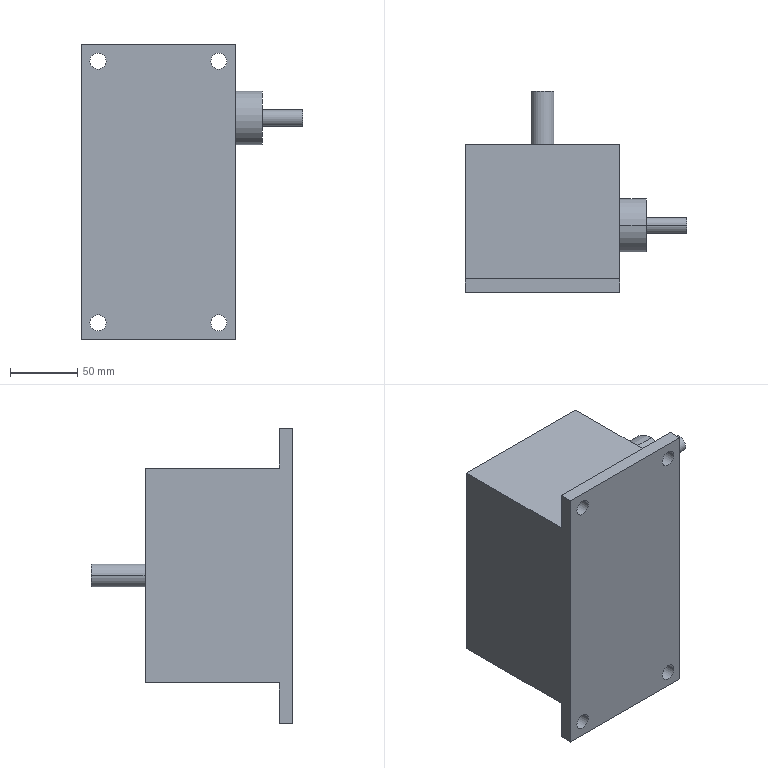Component | SolidWorks | Motor2-1 | 1 solid | 27 faces | box 165 x 150 x 220 mm | volume 2126081 mm3 | cylinder 14 | plane 13 | commonest cylinder face diameters 12 x10 40 x2 17 x2
build123d program:
from build123d import *

# Parameters (mm, degrees)
SKETCH1_W      = 220
SKETCH1_H      = 115
SKETCH1_R      = 6
EXTRUDE1_DEPTH = 10
SKETCH2_W      = 160
SKETCH2_H      = 115
EXTRUDE2_DEPTH = 100
SKETCH4_R      = 8.5
EXTRUDE3_DEPTH = 40
SKETCH5_R      = 20
EXTRUDE4_DEPTH = 20
SKETCH6_R      = 6
EXTRUDE5_DEPTH = 30


with BuildPart() as part:
    # Sketch1 → Extrude1 (new body)
    with BuildSketch(Plane(origin=(0, 0, 0), x_dir=(1, 0, 0), z_dir=(0, 1, 0))):
        with Locations((71.152, -39.253)):
            Rectangle(SKETCH1_W, SKETCH1_H)
        with Locations(Location((-26.348, 5.747, 0), (0, 0, 270))):
            Circle(SKETCH1_R, mode=Mode.SUBTRACT)
        with Locations(Location((168.652, 5.747, 0), (0, 0, 270))):
            Circle(SKETCH1_R, mode=Mode.SUBTRACT)
        with Locations(Location((-26.348, -84.253, 0), (0, 0, 270))):
            Circle(SKETCH1_R, mode=Mode.SUBTRACT)
        with Locations(Location((168.652, -84.253, 0), (0, 0, 270))):
            Circle(SKETCH1_R, mode=Mode.SUBTRACT)
    extrude(amount=EXTRUDE1_DEPTH)

    # Sketch2 → Extrude2 (add)
    with BuildSketch(Plane(origin=(0, 10, 0), x_dir=(1, 0, 0), z_dir=(0, 1, 0))):
        with Locations((70.757, -39.253)):
            Rectangle(SKETCH2_W, SKETCH2_H)
    extrude(amount=EXTRUDE2_DEPTH)

    # Sketch4 → Extrude3 (add)
    with BuildSketch(Plane(origin=(0, 110, 0), x_dir=(-1, 0, 0), z_dir=(0, 1, 0))):
        with Locations(Location((-70.757, 39.253, 0), (0, 0, 90))):
            Circle(SKETCH4_R)
    extrude(amount=EXTRUDE3_DEPTH)

    # Sketch5 → Extrude4 (add)
    with BuildSketch(Plane.XY.offset(96.753)):
        with Locations(Location((16.02, 50, 0), (0, 0, 180))):
            Circle(SKETCH5_R)
    extrude(amount=EXTRUDE4_DEPTH)

    # Sketch6 → Extrude5 (add)
    with BuildSketch(Plane.XY.offset(116.753)):
        with Locations((16.02, 50)):
            Circle(SKETCH6_R)
    extrude(amount=EXTRUDE5_DEPTH)


solid = part.part

# Placed as in the assembly
solid = solid.moved(Location((-204.037, 125.983, 74.757), (0, 90, 0)))
STEP:
#1=COLOUR_RGB('',0.7922,0.8196,0.9333);
#2=FILL_AREA_STYLE_COLOUR('',#1);
#3=FILL_AREA_STYLE('',(#2));
#4=SURFACE_STYLE_FILL_AREA(#3);
#5=SURFACE_SIDE_STYLE('',(#4));
#6=SURFACE_STYLE_USAGE(.BOTH.,#5);
#7=PRESENTATION_STYLE_ASSIGNMENT((#6));
#8=CARTESIAN_POINT('',(-2.255,6.928,2.076));
#9=VERTEX_POINT('',#8);
#10=CARTESIAN_POINT('',(-2.255,6.928,2.549));
#11=VERTEX_POINT('',#10);
#12=CARTESIAN_POINT('',(-2.255,6.928,2.312));
#13=DIRECTION('',(1.,0.,0.));
#14=DIRECTION('',(0.,0.,-1.));
#15=AXIS2_PLACEMENT_3D('',#12,#13,#14);
#16=CIRCLE('',#15,0.2362);
#17=EDGE_CURVE('',#9,#11,#16,.T.);
#18=ORIENTED_EDGE('',*,*,#17,.F.);
#19=CARTESIAN_POINT('',(-3.436,6.928,2.076));
#20=VERTEX_POINT('',#19);
#21=CARTESIAN_POINT('',(-2.255,6.928,2.076));
#22=DIRECTION('',(-1.,-0.,-0.));
#23=VECTOR('',#22,39.37);
#24=LINE('',#21,#23);
#25=EDGE_CURVE('',#9,#20,#24,.T.);
#26=ORIENTED_EDGE('',*,*,#25,.T.);
#27=CARTESIAN_POINT('',(-3.436,6.928,2.549));
#28=VERTEX_POINT('',#27);
#29=CARTESIAN_POINT('',(-3.436,6.928,2.312));
#30=DIRECTION('',(1.,0.,0.));
#31=DIRECTION('',(0.,0.,-1.));
#32=AXIS2_PLACEMENT_3D('',#29,#30,#31);
#33=CIRCLE('',#32,0.2362);
#34=EDGE_CURVE('',#20,#28,#33,.T.);
#35=ORIENTED_EDGE('',*,*,#34,.T.);
#36=CARTESIAN_POINT('',(-2.255,6.928,2.549));
#37=DIRECTION('',(-1.,-0.,-0.));
#38=VECTOR('',#37,39.37);
#39=LINE('',#36,#38);
#40=EDGE_CURVE('',#11,#28,#39,.T.);
#41=ORIENTED_EDGE('',*,*,#40,.F.);
#42=EDGE_LOOP('',(#18,#26,#35,#41));
#43=FACE_OUTER_BOUND('',#42,.T.);
#44=CARTESIAN_POINT('',(-2.255,6.928,2.312));
#45=DIRECTION('',(-1.,-0.,-0.));
#46=DIRECTION('',(0.,0.,1.));
#47=AXIS2_PLACEMENT_3D('',#44,#45,#46);
#48=CYLINDRICAL_SURFACE('',#47,0.2362);
#49=ADVANCED_FACE('',(#43),#48,.T.);
#50=CARTESIAN_POINT('',(-3.436,6.928,1.525));
#51=VERTEX_POINT('',#50);
#52=CARTESIAN_POINT('',(-3.436,6.928,3.1));
#53=VERTEX_POINT('',#52);
#54=CARTESIAN_POINT('',(-3.436,6.928,2.312));
#55=DIRECTION('',(1.,0.,0.));
#56=DIRECTION('',(0.,0.,-1.));
#57=AXIS2_PLACEMENT_3D('',#54,#55,#56);
#58=CIRCLE('',#57,0.7874);
#59=EDGE_CURVE('',#51,#53,#58,.T.);
#60=ORIENTED_EDGE('',*,*,#59,.F.);
#61=CARTESIAN_POINT('',(-4.224,6.928,1.525));
#62=VERTEX_POINT('',#61);
#63=CARTESIAN_POINT('',(-3.436,6.928,1.525));
#64=DIRECTION('',(-1.,-0.,-0.));
#65=VECTOR('',#64,39.37);
#66=LINE('',#63,#65);
#67=EDGE_CURVE('',#51,#62,#66,.T.);
#68=ORIENTED_EDGE('',*,*,#67,.T.);
#69=CARTESIAN_POINT('',(-4.224,6.928,3.1));
#70=VERTEX_POINT('',#69);
#71=CARTESIAN_POINT('',(-4.224,6.928,2.312));
#72=DIRECTION('',(1.,0.,0.));
#73=DIRECTION('',(0.,0.,1.));
#74=AXIS2_PLACEMENT_3D('',#71,#72,#73);
#75=CIRCLE('',#74,0.7874);
#76=EDGE_CURVE('',#62,#70,#75,.T.);
#77=ORIENTED_EDGE('',*,*,#76,.T.);
#78=CARTESIAN_POINT('',(-3.436,6.928,3.1));
#79=DIRECTION('',(-1.,-0.,-0.));
#80=VECTOR('',#79,39.37);
#81=LINE('',#78,#80);
#82=EDGE_CURVE('',#53,#70,#81,.T.);
#83=ORIENTED_EDGE('',*,*,#82,.F.);
#84=EDGE_LOOP('',(#60,#68,#77,#83));
#85=FACE_OUTER_BOUND('',#84,.T.);
#86=CARTESIAN_POINT('',(-3.436,6.928,2.312));
#87=DIRECTION('',(-1.,-0.,-0.));
#88=DIRECTION('',(0.,0.,1.));
#89=AXIS2_PLACEMENT_3D('',#86,#87,#88);
#90=CYLINDRICAL_SURFACE('',#89,0.7874);
#91=ADVANCED_FACE('',(#85),#90,.T.);
#92=CARTESIAN_POINT('',(-6.153,10.865,0.1575));
#93=VERTEX_POINT('',#92);
#94=CARTESIAN_POINT('',(-6.822,10.865,0.1575));
#95=VERTEX_POINT('',#94);
#96=CARTESIAN_POINT('',(-6.488,10.865,0.1575));
#97=DIRECTION('',(-0.,1.,-0.));
#98=DIRECTION('',(1.,0.,0.));
#99=AXIS2_PLACEMENT_3D('',#96,#97,#98);
#100=CIRCLE('',#99,0.3346);
#101=EDGE_CURVE('',#93,#95,#100,.T.);
#102=ORIENTED_EDGE('',*,*,#101,.F.);
#103=CARTESIAN_POINT('',(-6.153,9.291,0.1575));
#104=VERTEX_POINT('',#103);
#105=CARTESIAN_POINT('',(-6.153,10.865,0.1575));
#106=DIRECTION('',(0.,-1.,0.));
#107=VECTOR('',#106,39.37);
#108=LINE('',#105,#107);
#109=EDGE_CURVE('',#93,#104,#108,.T.);
#110=ORIENTED_EDGE('',*,*,#109,.T.);
#111=CARTESIAN_POINT('',(-6.822,9.291,0.1575));
#112=VERTEX_POINT('',#111);
#113=CARTESIAN_POINT('',(-6.488,9.291,0.1575));
#114=DIRECTION('',(-0.,1.,-0.));
#115=DIRECTION('',(1.,0.,0.));
#116=AXIS2_PLACEMENT_3D('',#113,#114,#115);
#117=CIRCLE('',#116,0.3346);
#118=EDGE_CURVE('',#104,#112,#117,.T.);
#119=ORIENTED_EDGE('',*,*,#118,.T.);
#120=CARTESIAN_POINT('',(-6.822,10.865,0.1575));
#121=DIRECTION('',(0.,-1.,0.));
#122=VECTOR('',#121,39.37);
#123=LINE('',#120,#122);
#124=EDGE_CURVE('',#95,#112,#123,.T.);
#125=ORIENTED_EDGE('',*,*,#124,.F.);
#126=EDGE_LOOP('',(#102,#110,#119,#125));
#127=FACE_OUTER_BOUND('',#126,.T.);
#128=CARTESIAN_POINT('',(-6.488,10.865,0.1575));
#129=DIRECTION('',(0.,-1.,0.));
#130=DIRECTION('',(-1.,0.,-0.));
#131=AXIS2_PLACEMENT_3D('',#128,#129,#130);
#132=CYLINDRICAL_SURFACE('',#131,0.3346);
#133=ADVANCED_FACE('',(#127),#132,.T.);
#134=CARTESIAN_POINT('',(-4.952,5.354,-3.697));
#135=VERTEX_POINT('',#134);
#136=CARTESIAN_POINT('',(-4.48,5.354,-3.697));
#137=VERTEX_POINT('',#136);
#138=CARTESIAN_POINT('',(-4.716,5.354,-3.697));
#139=DIRECTION('',(-0.,1.,-0.));
#140=DIRECTION('',(1.,0.,0.));
#141=AXIS2_PLACEMENT_3D('',#138,#139,#140);
#142=CIRCLE('',#141,0.2362);
#143=EDGE_CURVE('',#135,#137,#142,.T.);
#144=ORIENTED_EDGE('',*,*,#143,.T.);
#145=CARTESIAN_POINT('',(-4.48,4.96,-3.697));
#146=VERTEX_POINT('',#145);
#147=CARTESIAN_POINT('',(-4.48,5.354,-3.697));
#148=DIRECTION('',(0.,-1.,0.));
#149=VECTOR('',#148,39.37);
#150=LINE('',#147,#149);
#151=EDGE_CURVE('',#137,#146,#150,.T.);
#152=ORIENTED_EDGE('',*,*,#151,.T.);
#153=CARTESIAN_POINT('',(-4.952,4.96,-3.697));
#154=VERTEX_POINT('',#153);
#155=CARTESIAN_POINT('',(-4.716,4.96,-3.697));
#156=DIRECTION('',(-0.,1.,-0.));
#157=DIRECTION('',(1.,0.,0.));
#158=AXIS2_PLACEMENT_3D('',#155,#156,#157);
#159=CIRCLE('',#158,0.2362);
#160=EDGE_CURVE('',#154,#146,#159,.T.);
#161=ORIENTED_EDGE('',*,*,#160,.F.);
#162=CARTESIAN_POINT('',(-4.952,5.354,-3.697));
#163=DIRECTION('',(0.,-1.,0.));
#164=VECTOR('',#163,39.37);
#165=LINE('',#162,#164);
#166=EDGE_CURVE('',#135,#154,#165,.T.);
#167=ORIENTED_EDGE('',*,*,#166,.F.);
#168=EDGE_LOOP('',(#144,#152,#161,#167));
#169=FACE_OUTER_BOUND('',#168,.T.);
#170=CARTESIAN_POINT('',(-4.716,5.354,-3.697));
#171=DIRECTION('',(0.,-1.,0.));
#172=DIRECTION('',(-1.,0.,0.));
#173=AXIS2_PLACEMENT_3D('',#170,#171,#172);
#174=CYLINDRICAL_SURFACE('',#173,0.2362);
#175=ADVANCED_FACE('',(#169),#174,.F.);
#176=CARTESIAN_POINT('',(-4.952,5.354,3.98));
#177=VERTEX_POINT('',#176);
#178=CARTESIAN_POINT('',(-4.48,5.354,3.98));
#179=VERTEX_POINT('',#178);
#180=CARTESIAN_POINT('',(-4.716,5.354,3.98));
#181=DIRECTION('',(-0.,1.,-0.));
#182=DIRECTION('',(1.,0.,0.));
#183=AXIS2_PLACEMENT_3D('',#180,#181,#182);
#184=CIRCLE('',#183,0.2362);
#185=EDGE_CURVE('',#177,#179,#184,.T.);
#186=ORIENTED_EDGE('',*,*,#185,.T.);
#187=CARTESIAN_POINT('',(-4.48,4.96,3.98));
#188=VERTEX_POINT('',#187);
#189=CARTESIAN_POINT('',(-4.48,5.354,3.98));
#190=DIRECTION('',(0.,-1.,0.));
#191=VECTOR('',#190,39.37);
#192=LINE('',#189,#191);
#193=EDGE_CURVE('',#179,#188,#192,.T.);
#194=ORIENTED_EDGE('',*,*,#193,.T.);
#195=CARTESIAN_POINT('',(-4.952,4.96,3.98));
#196=VERTEX_POINT('',#195);
#197=CARTESIAN_POINT('',(-4.716,4.96,3.98));
#198=DIRECTION('',(-0.,1.,-0.));
#199=DIRECTION('',(1.,0.,0.));
#200=AXIS2_PLACEMENT_3D('',#197,#198,#199);
#201=CIRCLE('',#200,0.2362);
#202=EDGE_CURVE('',#196,#188,#201,.T.);
#203=ORIENTED_EDGE('',*,*,#202,.F.);
#204=CARTESIAN_POINT('',(-4.952,5.354,3.98));
#205=DIRECTION('',(0.,-1.,0.));
#206=VECTOR('',#205,39.37);
#207=LINE('',#204,#206);
#208=EDGE_CURVE('',#177,#196,#207,.T.);
#209=ORIENTED_EDGE('',*,*,#208,.F.);
#210=EDGE_LOOP('',(#186,#194,#203,#209));
#211=FACE_OUTER_BOUND('',#210,.T.);
#212=CARTESIAN_POINT('',(-4.716,5.354,3.98));
#213=DIRECTION('',(0.,-1.,0.));
#214=DIRECTION('',(-1.,0.,0.));
#215=AXIS2_PLACEMENT_3D('',#212,#213,#214);
#216=CYLINDRICAL_SURFACE('',#215,0.2362);
#217=ADVANCED_FACE('',(#211),#216,.F.);
#218=CARTESIAN_POINT('',(-8.495,5.354,-3.697));
#219=VERTEX_POINT('',#218);
#220=CARTESIAN_POINT('',(-8.023,5.354,-3.697));
#221=VERTEX_POINT('',#220);
#222=CARTESIAN_POINT('',(-8.259,5.354,-3.697));
#223=DIRECTION('',(-0.,1.,-0.));
#224=DIRECTION('',(1.,0.,0.));
#225=AXIS2_PLACEMENT_3D('',#222,#223,#224);
#226=CIRCLE('',#225,0.2362);
#227=EDGE_CURVE('',#219,#221,#226,.T.);
#228=ORIENTED_EDGE('',*,*,#227,.T.);
#229=CARTESIAN_POINT('',(-8.023,4.96,-3.697));
#230=VERTEX_POINT('',#229);
#231=CARTESIAN_POINT('',(-8.023,5.354,-3.697));
#232=DIRECTION('',(0.,-1.,0.));
#233=VECTOR('',#232,39.37);
#234=LINE('',#231,#233);
#235=EDGE_CURVE('',#221,#230,#234,.T.);
#236=ORIENTED_EDGE('',*,*,#235,.T.);
#237=CARTESIAN_POINT('',(-8.495,4.96,-3.697));
#238=VERTEX_POINT('',#237);
#239=CARTESIAN_POINT('',(-8.259,4.96,-3.697));
#240=DIRECTION('',(-0.,1.,-0.));
#241=DIRECTION('',(1.,0.,0.));
#242=AXIS2_PLACEMENT_3D('',#239,#240,#241);
#243=CIRCLE('',#242,0.2362);
#244=EDGE_CURVE('',#238,#230,#243,.T.);
#245=ORIENTED_EDGE('',*,*,#244,.F.);
#246=CARTESIAN_POINT('',(-8.495,5.354,-3.697));
#247=DIRECTION('',(0.,-1.,0.));
#248=VECTOR('',#247,39.37);
#249=LINE('',#246,#248);
#250=EDGE_CURVE('',#219,#238,#249,.T.);
#251=ORIENTED_EDGE('',*,*,#250,.F.);
#252=EDGE_LOOP('',(#228,#236,#245,#251));
#253=FACE_OUTER_BOUND('',#252,.T.);
#254=CARTESIAN_POINT('',(-8.259,5.354,-3.697));
#255=DIRECTION('',(0.,-1.,0.));
#256=DIRECTION('',(-1.,0.,0.));
#257=AXIS2_PLACEMENT_3D('',#254,#255,#256);
#258=CYLINDRICAL_SURFACE('',#257,0.2362);
#259=ADVANCED_FACE('',(#253),#258,.F.);
#260=CARTESIAN_POINT('',(-8.495,5.354,3.98));
#261=VERTEX_POINT('',#260);
#262=CARTESIAN_POINT('',(-8.023,5.354,3.98));
#263=VERTEX_POINT('',#262);
#264=CARTESIAN_POINT('',(-8.259,5.354,3.98));
#265=DIRECTION('',(-0.,1.,-0.));
#266=DIRECTION('',(1.,0.,0.));
#267=AXIS2_PLACEMENT_3D('',#264,#265,#266);
#268=CIRCLE('',#267,0.2362);
#269=EDGE_CURVE('',#261,#263,#268,.T.);
#270=ORIENTED_EDGE('',*,*,#269,.T.);
#271=CARTESIAN_POINT('',(-8.023,4.96,3.98));
#272=VERTEX_POINT('',#271);
#273=CARTESIAN_POINT('',(-8.023,5.354,3.98));
#274=DIRECTION('',(0.,-1.,0.));
#275=VECTOR('',#274,39.37);
#276=LINE('',#273,#275);
#277=EDGE_CURVE('',#263,#272,#276,.T.);
#278=ORIENTED_EDGE('',*,*,#277,.T.);
#279=CARTESIAN_POINT('',(-8.495,4.96,3.98));
#280=VERTEX_POINT('',#279);
#281=CARTESIAN_POINT('',(-8.259,4.96,3.98));
#282=DIRECTION('',(-0.,1.,-0.));
#283=DIRECTION('',(1.,0.,0.));
#284=AXIS2_PLACEMENT_3D('',#281,#282,#283);
#285=CIRCLE('',#284,0.2362);
#286=EDGE_CURVE('',#280,#272,#285,.T.);
#287=ORIENTED_EDGE('',*,*,#286,.F.);
#288=CARTESIAN_POINT('',(-8.495,5.354,3.98));
#289=DIRECTION('',(0.,-1.,0.));
#290=VECTOR('',#289,39.37);
#291=LINE('',#288,#290);
#292=EDGE_CURVE('',#261,#280,#291,.T.);
#293=ORIENTED_EDGE('',*,*,#292,.F.);
#294=EDGE_LOOP('',(#270,#278,#287,#293));
#295=FACE_OUTER_BOUND('',#294,.T.);
#296=CARTESIAN_POINT('',(-8.259,5.354,3.98));
#297=DIRECTION('',(0.,-1.,0.));
#298=DIRECTION('',(-1.,0.,0.));
#299=AXIS2_PLACEMENT_3D('',#296,#297,#298);
#300=CYLINDRICAL_SURFACE('',#299,0.2362);
#301=ADVANCED_FACE('',(#295),#300,.F.);
#302=CARTESIAN_POINT('',(-3.436,6.928,2.312));
#303=DIRECTION('',(1.,0.,0.));
#304=DIRECTION('',(0.,0.,-1.));
#305=AXIS2_PLACEMENT_3D('',#302,#303,#304);
#306=CIRCLE('',#305,0.7874);
#307=EDGE_CURVE('',#53,#51,#306,.T.);
#308=ORIENTED_EDGE('',*,*,#307,.T.);
#309=ORIENTED_EDGE('',*,*,#59,.T.);
#310=EDGE_LOOP('',(#308,#309));
#311=FACE_OUTER_BOUND('',#310,.T.);
#312=CARTESIAN_POINT('',(-3.436,6.928,2.312));
#313=DIRECTION('',(1.,0.,0.));
#314=DIRECTION('',(0.,0.,-1.));
#315=AXIS2_PLACEMENT_3D('',#312,#313,#314);
#316=CIRCLE('',#315,0.2362);
#317=EDGE_CURVE('',#28,#20,#316,.T.);
#318=ORIENTED_EDGE('',*,*,#317,.F.);
#319=ORIENTED_EDGE('',*,*,#34,.F.);
#320=EDGE_LOOP('',(#318,#319));
#321=FACE_BOUND('',#320,.T.);
#322=CARTESIAN_POINT('',(-3.436,6.928,2.312));
#323=DIRECTION('',(1.,0.,0.));
#324=DIRECTION('',(0.,-0.,-1.));
#325=AXIS2_PLACEMENT_3D('',#322,#323,#324);
#326=PLANE('',#325);
#327=ADVANCED_FACE('',(#311,#321),#326,.T.);
#328=CARTESIAN_POINT('',(-4.224,4.96,4.473));
#329=VERTEX_POINT('',#328);
#330=CARTESIAN_POINT('',(-4.224,4.96,-4.189));
#331=VERTEX_POINT('',#330);
#332=CARTESIAN_POINT('',(-4.224,4.96,4.473));
#333=DIRECTION('',(0.,-0.,-1.));
#334=VECTOR('',#333,39.37);
#335=LINE('',#332,#334);
#336=EDGE_CURVE('',#329,#331,#335,.T.);
#337=ORIENTED_EDGE('',*,*,#336,.T.);
#338=CARTESIAN_POINT('',(-4.224,5.354,-4.189));
#339=VERTEX_POINT('',#338);
#340=CARTESIAN_POINT('',(-4.224,5.354,-4.189));
#341=DIRECTION('',(0.,-1.,0.));
#342=VECTOR('',#341,39.37);
#343=LINE('',#340,#342);
#344=EDGE_CURVE('',#339,#331,#343,.T.);
#345=ORIENTED_EDGE('',*,*,#344,.F.);
#346=CARTESIAN_POINT('',(-4.224,5.354,-2.992));
#347=VERTEX_POINT('',#346);
#348=CARTESIAN_POINT('',(-4.224,5.354,4.473));
#349=DIRECTION('',(0.,-0.,-1.));
#350=VECTOR('',#349,39.37);
#351=LINE('',#348,#350);
#352=EDGE_CURVE('',#347,#339,#351,.T.);
#353=ORIENTED_EDGE('',*,*,#352,.F.);
#354=CARTESIAN_POINT('',(-4.224,9.291,-2.992));
#355=VERTEX_POINT('',#354);
#356=CARTESIAN_POINT('',(-4.224,9.291,-2.992));
#357=DIRECTION('',(0.,-1.,0.));
#358=VECTOR('',#357,39.37);
#359=LINE('',#356,#358);
#360=EDGE_CURVE('',#355,#347,#359,.T.);
#361=ORIENTED_EDGE('',*,*,#360,.F.);
#362=CARTESIAN_POINT('',(-4.224,9.291,3.307));
#363=VERTEX_POINT('',#362);
#364=CARTESIAN_POINT('',(-4.224,9.291,3.307));
#365=DIRECTION('',(0.,-0.,-1.));
#366=VECTOR('',#365,39.37);
#367=LINE('',#364,#366);
#368=EDGE_CURVE('',#363,#355,#367,.T.);
#369=ORIENTED_EDGE('',*,*,#368,.F.);
#370=CARTESIAN_POINT('',(-4.224,5.354,3.307));
#371=VERTEX_POINT('',#370);
#372=CARTESIAN_POINT('',(-4.224,9.291,3.307));
#373=DIRECTION('',(0.,-1.,0.));
#374=VECTOR('',#373,39.37);
#375=LINE('',#372,#374);
#376=EDGE_CURVE('',#363,#371,#375,.T.);
#377=ORIENTED_EDGE('',*,*,#376,.T.);
#378=CARTESIAN_POINT('',(-4.224,5.354,4.473));
#379=VERTEX_POINT('',#378);
#380=CARTESIAN_POINT('',(-4.224,5.354,4.473));
#381=DIRECTION('',(0.,-0.,-1.));
#382=VECTOR('',#381,39.37);
#383=LINE('',#380,#382);
#384=EDGE_CURVE('',#379,#371,#383,.T.);
#385=ORIENTED_EDGE('',*,*,#384,.F.);
#386=CARTESIAN_POINT('',(-4.224,5.354,4.473));
#387=DIRECTION('',(0.,-1.,0.));
#388=VECTOR('',#387,39.37);
#389=LINE('',#386,#388);
#390=EDGE_CURVE('',#379,#329,#389,.T.);
#391=ORIENTED_EDGE('',*,*,#390,.T.);
#392=EDGE_LOOP('',(#337,#345,#353,#361,#369,#377,#385,#391));
#393=FACE_OUTER_BOUND('',#392,.T.);
#394=CARTESIAN_POINT('',(-4.224,6.928,2.312));
#395=DIRECTION('',(1.,0.,0.));
#396=DIRECTION('',(0.,0.,1.));
#397=AXIS2_PLACEMENT_3D('',#394,#395,#396);
#398=CIRCLE('',#397,0.7874);
#399=EDGE_CURVE('',#70,#62,#398,.T.);
#400=ORIENTED_EDGE('',*,*,#399,.F.);
#401=ORIENTED_EDGE('',*,*,#76,.F.);
#402=EDGE_LOOP('',(#400,#401));
#403=FACE_BOUND('',#402,.T.);
#404=CARTESIAN_POINT('',(-4.224,5.354,4.473));
#405=DIRECTION('',(-1.,-0.,-0.));
#406=DIRECTION('',(-0.,0.,1.));
#407=AXIS2_PLACEMENT_3D('',#404,#405,#406);
#408=PLANE('',#407);
#409=ADVANCED_FACE('',(#393,#403),#408,.F.);
#410=CARTESIAN_POINT('',(-8.751,9.291,3.307));
#411=VERTEX_POINT('',#410);
#412=CARTESIAN_POINT('',(-8.751,9.291,3.307));
#413=DIRECTION('',(1.,0.,0.));
#414=VECTOR('',#413,39.37);
#415=LINE('',#412,#414);
#416=EDGE_CURVE('',#411,#363,#415,.T.);
#417=ORIENTED_EDGE('',*,*,#416,.T.);
#418=ORIENTED_EDGE('',*,*,#368,.T.);
#419=CARTESIAN_POINT('',(-8.751,9.291,-2.992));
#420=VERTEX_POINT('',#419);
#421=CARTESIAN_POINT('',(-8.751,9.291,-2.992));
#422=DIRECTION('',(-1.,-0.,-0.));
#423=VECTOR('',#422,39.37);
#424=LINE('',#421,#423);
#425=EDGE_CURVE('',#355,#420,#424,.T.);
#426=ORIENTED_EDGE('',*,*,#425,.T.);
#427=CARTESIAN_POINT('',(-8.751,9.291,3.307));
#428=DIRECTION('',(-0.,0.,1.));
#429=VECTOR('',#428,39.37);
#430=LINE('',#427,#429);
#431=EDGE_CURVE('',#420,#411,#430,.T.);
#432=ORIENTED_EDGE('',*,*,#431,.T.);
#433=EDGE_LOOP('',(#417,#418,#426,#432));
#434=FACE_OUTER_BOUND('',#433,.T.);
#435=CARTESIAN_POINT('',(-6.488,9.291,0.1575));
#436=DIRECTION('',(-0.,1.,-0.));
#437=DIRECTION('',(1.,0.,0.));
#438=AXIS2_PLACEMENT_3D('',#435,#436,#437);
#439=CIRCLE('',#438,0.3346);
#440=EDGE_CURVE('',#112,#104,#439,.T.);
#441=ORIENTED_EDGE('',*,*,#440,.F.);
#442=ORIENTED_EDGE('',*,*,#118,.F.);
#443=EDGE_LOOP('',(#441,#442));
#444=FACE_BOUND('',#443,.T.);
#445=CARTESIAN_POINT('',(-4.224,9.291,3.307));
#446=DIRECTION('',(-0.,1.,-0.));
#447=DIRECTION('',(1.,0.,0.));
#448=AXIS2_PLACEMENT_3D('',#445,#446,#447);
#449=PLANE('',#448);
#450=ADVANCED_FACE('',(#434,#444),#449,.T.);
#451=CARTESIAN_POINT('',(-8.751,5.354,3.307));
#452=VERTEX_POINT('',#451);
#453=CARTESIAN_POINT('',(-8.751,5.354,3.307));
#454=DIRECTION('',(1.,0.,0.));
#455=VECTOR('',#454,39.37);
#456=LINE('',#453,#455);
#457=EDGE_CURVE('',#452,#371,#456,.T.);
#458=ORIENTED_EDGE('',*,*,#457,.F.);
#459=CARTESIAN_POINT('',(-8.751,5.354,4.473));
#460=VERTEX_POINT('',#459);
#461=CARTESIAN_POINT('',(-8.751,5.354,4.473));
#462=DIRECTION('',(-0.,0.,1.));
#463=VECTOR('',#462,39.37);
#464=LINE('',#461,#463);
#465=EDGE_CURVE('',#452,#460,#464,.T.);
#466=ORIENTED_EDGE('',*,*,#465,.T.);
#467=CARTESIAN_POINT('',(-8.751,5.354,4.473));
#468=DIRECTION('',(1.,0.,-0.));
#469=VECTOR('',#468,39.37);
#470=LINE('',#467,#469);
#471=EDGE_CURVE('',#460,#379,#470,.T.);
#472=ORIENTED_EDGE('',*,*,#471,.T.);
#473=ORIENTED_EDGE('',*,*,#384,.T.);
#474=EDGE_LOOP('',(#458,#466,#472,#473));
#475=FACE_OUTER_BOUND('',#474,.T.);
#476=ORIENTED_EDGE('',*,*,#269,.F.);
#477=CARTESIAN_POINT('',(-8.259,5.354,3.98));
#478=DIRECTION('',(-0.,1.,-0.));
#479=DIRECTION('',(1.,0.,0.));
#480=AXIS2_PLACEMENT_3D('',#477,#478,#479);
#481=CIRCLE('',#480,0.2362);
#482=EDGE_CURVE('',#263,#261,#481,.T.);
#483=ORIENTED_EDGE('',*,*,#482,.F.);
#484=EDGE_LOOP('',(#476,#483));
#485=FACE_BOUND('',#484,.T.);
#486=ORIENTED_EDGE('',*,*,#185,.F.);
#487=CARTESIAN_POINT('',(-4.716,5.354,3.98));
#488=DIRECTION('',(-0.,1.,-0.));
#489=DIRECTION('',(1.,0.,0.));
#490=AXIS2_PLACEMENT_3D('',#487,#488,#489);
#491=CIRCLE('',#490,0.2362);
#492=EDGE_CURVE('',#179,#177,#491,.T.);
#493=ORIENTED_EDGE('',*,*,#492,.F.);
#494=EDGE_LOOP('',(#486,#493));
#495=FACE_BOUND('',#494,.T.);
#496=CARTESIAN_POINT('',(-4.224,5.354,4.473));
#497=DIRECTION('',(-0.,1.,-0.));
#498=DIRECTION('',(1.,0.,0.));
#499=AXIS2_PLACEMENT_3D('',#496,#497,#498);
#500=PLANE('',#499);
#501=ADVANCED_FACE('',(#475,#485,#495),#500,.T.);
#502=CARTESIAN_POINT('',(-8.751,5.354,-2.992));
#503=VERTEX_POINT('',#502);
#504=CARTESIAN_POINT('',(-8.751,5.354,-2.992));
#505=DIRECTION('',(-1.,-0.,-0.));
#506=VECTOR('',#505,39.37);
#507=LINE('',#504,#506);
#508=EDGE_CURVE('',#347,#503,#507,.T.);
#509=ORIENTED_EDGE('',*,*,#508,.F.);
#510=ORIENTED_EDGE('',*,*,#352,.T.);
#511=CARTESIAN_POINT('',(-8.751,5.354,-4.189));
#512=VERTEX_POINT('',#511);
#513=CARTESIAN_POINT('',(-8.751,5.354,-4.189));
#514=DIRECTION('',(-1.,-0.,0.));
#515=VECTOR('',#514,39.37);
#516=LINE('',#513,#515);
#517=EDGE_CURVE('',#339,#512,#516,.T.);
#518=ORIENTED_EDGE('',*,*,#517,.T.);
#519=CARTESIAN_POINT('',(-8.751,5.354,4.473));
#520=DIRECTION('',(-0.,0.,1.));
#521=VECTOR('',#520,39.37);
#522=LINE('',#519,#521);
#523=EDGE_CURVE('',#512,#503,#522,.T.);
#524=ORIENTED_EDGE('',*,*,#523,.T.);
#525=EDGE_LOOP('',(#509,#510,#518,#524));
#526=FACE_OUTER_BOUND('',#525,.T.);
#527=ORIENTED_EDGE('',*,*,#227,.F.);
#528=CARTESIAN_POINT('',(-8.259,5.354,-3.697));
#529=DIRECTION('',(-0.,1.,-0.));
#530=DIRECTION('',(1.,0.,0.));
#531=AXIS2_PLACEMENT_3D('',#528,#529,#530);
#532=CIRCLE('',#531,0.2362);
#533=EDGE_CURVE('',#221,#219,#532,.T.);
#534=ORIENTED_EDGE('',*,*,#533,.F.);
#535=EDGE_LOOP('',(#527,#534));
#536=FACE_BOUND('',#535,.T.);
#537=ORIENTED_EDGE('',*,*,#143,.F.);
#538=CARTESIAN_POINT('',(-4.716,5.354,-3.697));
#539=DIRECTION('',(-0.,1.,-0.));
#540=DIRECTION('',(1.,0.,0.));
#541=AXIS2_PLACEMENT_3D('',#538,#539,#540);
#542=CIRCLE('',#541,0.2362);
#543=EDGE_CURVE('',#137,#135,#542,.T.);
#544=ORIENTED_EDGE('',*,*,#543,.F.);
#545=EDGE_LOOP('',(#537,#544));
#546=FACE_BOUND('',#545,.T.);
#547=CARTESIAN_POINT('',(-4.224,5.354,4.473));
#548=DIRECTION('',(-0.,1.,-0.));
#549=DIRECTION('',(1.,0.,0.));
#550=AXIS2_PLACEMENT_3D('',#547,#548,#549);
#551=PLANE('',#550);
#552=ADVANCED_FACE('',(#526,#536,#546),#551,.T.);
#553=CARTESIAN_POINT('',(-8.751,4.96,4.473));
#554=VERTEX_POINT('',#553);
#555=CARTESIAN_POINT('',(-8.751,4.96,4.473));
#556=DIRECTION('',(1.,0.,-0.));
#557=VECTOR('',#556,39.37);
#558=LINE('',#555,#557);
#559=EDGE_CURVE('',#554,#329,#558,.T.);
#560=ORIENTED_EDGE('',*,*,#559,.F.);
#561=CARTESIAN_POINT('',(-8.751,4.96,-4.189));
#562=VERTEX_POINT('',#561);
#563=CARTESIAN_POINT('',(-8.751,4.96,4.473));
#564=DIRECTION('',(-0.,0.,1.));
#565=VECTOR('',#564,39.37);
#566=LINE('',#563,#565);
#567=EDGE_CURVE('',#562,#554,#566,.T.);
#568=ORIENTED_EDGE('',*,*,#567,.F.);
#569=CARTESIAN_POINT('',(-8.751,4.96,-4.189));
#570=DIRECTION('',(-1.,-0.,0.));
#571=VECTOR('',#570,39.37);
#572=LINE('',#569,#571);
#573=EDGE_CURVE('',#331,#562,#572,.T.);
#574=ORIENTED_EDGE('',*,*,#573,.F.);
#575=ORIENTED_EDGE('',*,*,#336,.F.);
#576=EDGE_LOOP('',(#560,#568,#574,#575));
#577=FACE_OUTER_BOUND('',#576,.T.);
#578=ORIENTED_EDGE('',*,*,#286,.T.);
#579=CARTESIAN_POINT('',(-8.259,4.96,3.98));
#580=DIRECTION('',(-0.,1.,-0.));
#581=DIRECTION('',(1.,0.,0.));
#582=AXIS2_PLACEMENT_3D('',#579,#580,#581);
#583=CIRCLE('',#582,0.2362);
#584=EDGE_CURVE('',#272,#280,#583,.T.);
#585=ORIENTED_EDGE('',*,*,#584,.T.);
#586=EDGE_LOOP('',(#578,#585));
#587=FACE_BOUND('',#586,.T.);
#588=ORIENTED_EDGE('',*,*,#244,.T.);
#589=CARTESIAN_POINT('',(-8.259,4.96,-3.697));
#590=DIRECTION('',(-0.,1.,-0.));
#591=DIRECTION('',(1.,0.,0.));
#592=AXIS2_PLACEMENT_3D('',#589,#590,#591);
#593=CIRCLE('',#592,0.2362);
#594=EDGE_CURVE('',#230,#238,#593,.T.);
#595=ORIENTED_EDGE('',*,*,#594,.T.);
#596=EDGE_LOOP('',(#588,#595));
#597=FACE_BOUND('',#596,.T.);
#598=ORIENTED_EDGE('',*,*,#202,.T.);
#599=CARTESIAN_POINT('',(-4.716,4.96,3.98));
#600=DIRECTION('',(-0.,1.,-0.));
#601=DIRECTION('',(1.,0.,0.));
#602=AXIS2_PLACEMENT_3D('',#599,#600,#601);
#603=CIRCLE('',#602,0.2362);
#604=EDGE_CURVE('',#188,#196,#603,.T.);
#605=ORIENTED_EDGE('',*,*,#604,.T.);
#606=EDGE_LOOP('',(#598,#605));
#607=FACE_BOUND('',#606,.T.);
#608=ORIENTED_EDGE('',*,*,#160,.T.);
#609=CARTESIAN_POINT('',(-4.716,4.96,-3.697));
#610=DIRECTION('',(-0.,1.,-0.));
#611=DIRECTION('',(1.,0.,0.));
#612=AXIS2_PLACEMENT_3D('',#609,#610,#611);
#613=CIRCLE('',#612,0.2362);
#614=EDGE_CURVE('',#146,#154,#613,.T.);
#615=ORIENTED_EDGE('',*,*,#614,.T.);
#616=EDGE_LOOP('',(#608,#615));
#617=FACE_BOUND('',#616,.T.);
#618=CARTESIAN_POINT('',(-4.224,4.96,4.473));
#619=DIRECTION('',(-0.,1.,-0.));
#620=DIRECTION('',(1.,0.,0.));
#621=AXIS2_PLACEMENT_3D('',#618,#619,#620);
#622=PLANE('',#621);
#623=ADVANCED_FACE('',(#577,#587,#597,#607,#617),#622,.F.);
#624=ORIENTED_EDGE('',*,*,#559,.T.);
#625=ORIENTED_EDGE('',*,*,#390,.F.);
#626=ORIENTED_EDGE('',*,*,#471,.F.);
#627=CARTESIAN_POINT('',(-8.751,5.354,4.473));
#628=DIRECTION('',(0.,-1.,0.));
#629=VECTOR('',#628,39.37);
#630=LINE('',#627,#629);
#631=EDGE_CURVE('',#460,#554,#630,.T.);
#632=ORIENTED_EDGE('',*,*,#631,.T.);
#633=EDGE_LOOP('',(#624,#625,#626,#632));
#634=FACE_OUTER_BOUND('',#633,.T.);
#635=CARTESIAN_POINT('',(-8.751,5.354,4.473));
#636=DIRECTION('',(-0.,-0.,-1.));
#637=DIRECTION('',(-1.,-0.,0.));
#638=AXIS2_PLACEMENT_3D('',#635,#636,#637);
#639=PLANE('',#638);
#640=ADVANCED_FACE('',(#634),#639,.F.);
#641=ORIENTED_EDGE('',*,*,#573,.T.);
#642=CARTESIAN_POINT('',(-8.751,5.354,-4.189));
#643=DIRECTION('',(0.,-1.,0.));
#644=VECTOR('',#643,39.37);
#645=LINE('',#642,#644);
#646=EDGE_CURVE('',#512,#562,#645,.T.);
#647=ORIENTED_EDGE('',*,*,#646,.F.);
#648=ORIENTED_EDGE('',*,*,#517,.F.);
#649=ORIENTED_EDGE('',*,*,#344,.T.);
#650=EDGE_LOOP('',(#641,#647,#648,#649));
#651=FACE_OUTER_BOUND('',#650,.T.);
#652=CARTESIAN_POINT('',(-8.751,5.354,-4.189));
#653=DIRECTION('',(0.,0.,1.));
#654=DIRECTION('',(1.,0.,-0.));
#655=AXIS2_PLACEMENT_3D('',#652,#653,#654);
#656=PLANE('',#655);
#657=ADVANCED_FACE('',(#651),#656,.F.);
#658=ORIENTED_EDGE('',*,*,#567,.T.);
#659=ORIENTED_EDGE('',*,*,#631,.F.);
#660=ORIENTED_EDGE('',*,*,#465,.F.);
#661=CARTESIAN_POINT('',(-8.751,9.291,3.307));
#662=DIRECTION('',(0.,-1.,0.));
#663=VECTOR('',#662,39.37);
#664=LINE('',#661,#663);
#665=EDGE_CURVE('',#411,#452,#664,.T.);
#666=ORIENTED_EDGE('',*,*,#665,.F.);
#667=ORIENTED_EDGE('',*,*,#431,.F.);
#668=CARTESIAN_POINT('',(-8.751,9.291,-2.992));
#669=DIRECTION('',(0.,-1.,0.));
#670=VECTOR('',#669,39.37);
#671=LINE('',#668,#670);
#672=EDGE_CURVE('',#420,#503,#671,.T.);
#673=ORIENTED_EDGE('',*,*,#672,.T.);
#674=ORIENTED_EDGE('',*,*,#523,.F.);
#675=ORIENTED_EDGE('',*,*,#646,.T.);
#676=EDGE_LOOP('',(#658,#659,#660,#666,#667,#673,#674,#675));
#677=FACE_OUTER_BOUND('',#676,.T.);
#678=CARTESIAN_POINT('',(-8.751,5.354,4.473));
#679=DIRECTION('',(1.,0.,0.));
#680=DIRECTION('',(0.,-0.,-1.));
#681=AXIS2_PLACEMENT_3D('',#678,#679,#680);
#682=PLANE('',#681);
#683=ADVANCED_FACE('',(#677),#682,.F.);
#684=ORIENTED_EDGE('',*,*,#277,.F.);
#685=ORIENTED_EDGE('',*,*,#482,.T.);
#686=ORIENTED_EDGE('',*,*,#292,.T.);
#687=ORIENTED_EDGE('',*,*,#584,.F.);
#688=EDGE_LOOP('',(#684,#685,#686,#687));
#689=FACE_OUTER_BOUND('',#688,.T.);
#690=CARTESIAN_POINT('',(-8.259,5.354,3.98));
#691=DIRECTION('',(0.,-1.,0.));
#692=DIRECTION('',(-1.,0.,0.));
#693=AXIS2_PLACEMENT_3D('',#690,#691,#692);
#694=CYLINDRICAL_SURFACE('',#693,0.2362);
#695=ADVANCED_FACE('',(#689),#694,.F.);
#696=ORIENTED_EDGE('',*,*,#235,.F.);
#697=ORIENTED_EDGE('',*,*,#533,.T.);
#698=ORIENTED_EDGE('',*,*,#250,.T.);
#699=ORIENTED_EDGE('',*,*,#594,.F.);
#700=EDGE_LOOP('',(#696,#697,#698,#699));
#701=FACE_OUTER_BOUND('',#700,.T.);
#702=CARTESIAN_POINT('',(-8.259,5.354,-3.697));
#703=DIRECTION('',(0.,-1.,0.));
#704=DIRECTION('',(-1.,0.,0.));
#705=AXIS2_PLACEMENT_3D('',#702,#703,#704);
#706=CYLINDRICAL_SURFACE('',#705,0.2362);
#707=ADVANCED_FACE('',(#701),#706,.F.);
#708=ORIENTED_EDGE('',*,*,#193,.F.);
#709=ORIENTED_EDGE('',*,*,#492,.T.);
#710=ORIENTED_EDGE('',*,*,#208,.T.);
#711=ORIENTED_EDGE('',*,*,#604,.F.);
#712=EDGE_LOOP('',(#708,#709,#710,#711));
#713=FACE_OUTER_BOUND('',#712,.T.);
#714=CARTESIAN_POINT('',(-4.716,5.354,3.98));
#715=DIRECTION('',(0.,-1.,0.));
#716=DIRECTION('',(-1.,0.,0.));
#717=AXIS2_PLACEMENT_3D('',#714,#715,#716);
#718=CYLINDRICAL_SURFACE('',#717,0.2362);
#719=ADVANCED_FACE('',(#713),#718,.F.);
#720=ORIENTED_EDGE('',*,*,#151,.F.);
#721=ORIENTED_EDGE('',*,*,#543,.T.);
#722=ORIENTED_EDGE('',*,*,#166,.T.);
#723=ORIENTED_EDGE('',*,*,#614,.F.);
#724=EDGE_LOOP('',(#720,#721,#722,#723));
#725=FACE_OUTER_BOUND('',#724,.T.);
#726=CARTESIAN_POINT('',(-4.716,5.354,-3.697));
#727=DIRECTION('',(0.,-1.,0.));
#728=DIRECTION('',(-1.,0.,0.));
#729=AXIS2_PLACEMENT_3D('',#726,#727,#728);
#730=CYLINDRICAL_SURFACE('',#729,0.2362);
#731=ADVANCED_FACE('',(#725),#730,.F.);
#732=ORIENTED_EDGE('',*,*,#457,.T.);
#733=ORIENTED_EDGE('',*,*,#376,.F.);
#734=ORIENTED_EDGE('',*,*,#416,.F.);
#735=ORIENTED_EDGE('',*,*,#665,.T.);
#736=EDGE_LOOP('',(#732,#733,#734,#735));
#737=FACE_OUTER_BOUND('',#736,.T.);
#738=CARTESIAN_POINT('',(-8.751,9.291,3.307));
#739=DIRECTION('',(0.,-0.,-1.));
#740=DIRECTION('',(-1.,-0.,-0.));
#741=AXIS2_PLACEMENT_3D('',#738,#739,#740);
#742=PLANE('',#741);
#743=ADVANCED_FACE('',(#737),#742,.F.);
#744=ORIENTED_EDGE('',*,*,#508,.T.);
#745=ORIENTED_EDGE('',*,*,#672,.F.);
#746=ORIENTED_EDGE('',*,*,#425,.F.);
#747=ORIENTED_EDGE('',*,*,#360,.T.);
#748=EDGE_LOOP('',(#744,#745,#746,#747));
#749=FACE_OUTER_BOUND('',#748,.T.);
#750=CARTESIAN_POINT('',(-8.751,9.291,-2.992));
#751=DIRECTION('',(-0.,0.,1.));
#752=DIRECTION('',(1.,0.,0.));
#753=AXIS2_PLACEMENT_3D('',#750,#751,#752);
#754=PLANE('',#753);
#755=ADVANCED_FACE('',(#749),#754,.F.);
#756=ORIENTED_EDGE('',*,*,#109,.F.);
#757=CARTESIAN_POINT('',(-6.488,10.865,0.1575));
#758=DIRECTION('',(-0.,1.,-0.));
#759=DIRECTION('',(1.,0.,0.));
#760=AXIS2_PLACEMENT_3D('',#757,#758,#759);
#761=CIRCLE('',#760,0.3346);
#762=EDGE_CURVE('',#95,#93,#761,.T.);
#763=ORIENTED_EDGE('',*,*,#762,.F.);
#764=ORIENTED_EDGE('',*,*,#124,.T.);
#765=ORIENTED_EDGE('',*,*,#440,.T.);
#766=EDGE_LOOP('',(#756,#763,#764,#765));
#767=FACE_OUTER_BOUND('',#766,.T.);
#768=CARTESIAN_POINT('',(-6.488,10.865,0.1575));
#769=DIRECTION('',(0.,-1.,0.));
#770=DIRECTION('',(-1.,0.,-0.));
#771=AXIS2_PLACEMENT_3D('',#768,#769,#770);
#772=CYLINDRICAL_SURFACE('',#771,0.3346);
#773=ADVANCED_FACE('',(#767),#772,.T.);
#774=ORIENTED_EDGE('',*,*,#762,.T.);
#775=ORIENTED_EDGE('',*,*,#101,.T.);
#776=EDGE_LOOP('',(#774,#775));
#777=FACE_OUTER_BOUND('',#776,.T.);
#778=CARTESIAN_POINT('',(-6.488,10.865,0.1575));
#779=DIRECTION('',(-0.,1.,-0.));
#780=DIRECTION('',(1.,0.,0.));
#781=AXIS2_PLACEMENT_3D('',#778,#779,#780);
#782=PLANE('',#781);
#783=ADVANCED_FACE('',(#777),#782,.T.);
#784=ORIENTED_EDGE('',*,*,#67,.F.);
#785=ORIENTED_EDGE('',*,*,#307,.F.);
#786=ORIENTED_EDGE('',*,*,#82,.T.);
#787=ORIENTED_EDGE('',*,*,#399,.T.);
#788=EDGE_LOOP('',(#784,#785,#786,#787));
#789=FACE_OUTER_BOUND('',#788,.T.);
#790=CARTESIAN_POINT('',(-3.436,6.928,2.312));
#791=DIRECTION('',(-1.,-0.,-0.));
#792=DIRECTION('',(0.,0.,1.));
#793=AXIS2_PLACEMENT_3D('',#790,#791,#792);
#794=CYLINDRICAL_SURFACE('',#793,0.7874);
#795=ADVANCED_FACE('',(#789),#794,.T.);
#796=ORIENTED_EDGE('',*,*,#25,.F.);
#797=CARTESIAN_POINT('',(-2.255,6.928,2.312));
#798=DIRECTION('',(1.,0.,0.));
#799=DIRECTION('',(0.,0.,-1.));
#800=AXIS2_PLACEMENT_3D('',#797,#798,#799);
#801=CIRCLE('',#800,0.2362);
#802=EDGE_CURVE('',#11,#9,#801,.T.);
#803=ORIENTED_EDGE('',*,*,#802,.F.);
#804=ORIENTED_EDGE('',*,*,#40,.T.);
#805=ORIENTED_EDGE('',*,*,#317,.T.);
#806=EDGE_LOOP('',(#796,#803,#804,#805));
#807=FACE_OUTER_BOUND('',#806,.T.);
#808=CARTESIAN_POINT('',(-2.255,6.928,2.312));
#809=DIRECTION('',(-1.,-0.,-0.));
#810=DIRECTION('',(0.,0.,1.));
#811=AXIS2_PLACEMENT_3D('',#808,#809,#810);
#812=CYLINDRICAL_SURFACE('',#811,0.2362);
#813=ADVANCED_FACE('',(#807),#812,.T.);
#814=ORIENTED_EDGE('',*,*,#802,.T.);
#815=ORIENTED_EDGE('',*,*,#17,.T.);
#816=EDGE_LOOP('',(#814,#815));
#817=FACE_OUTER_BOUND('',#816,.T.);
#818=CARTESIAN_POINT('',(-2.255,6.928,2.312));
#819=DIRECTION('',(1.,0.,0.));
#820=DIRECTION('',(0.,-0.,-1.));
#821=AXIS2_PLACEMENT_3D('',#818,#819,#820);
#822=PLANE('',#821);
#823=ADVANCED_FACE('',(#817),#822,.T.);
#824=CLOSED_SHELL('',(#49,#91,#133,#175,#217,#259,#301,#327,#409,#450,#501,#552,#623,#640,#657,#683,#695,#707,#719,#731,#743,#755,#773,#783,#795,#813,#823));
#825=MANIFOLD_SOLID_BREP('',#824);
#826=STYLED_ITEM('',(#7),#825);
#827=PRESENTATION_LAYER_ASSIGNMENT('','',(#826));
#828=(LENGTH_UNIT()NAMED_UNIT(*)SI_UNIT($,.METRE.));
#829=LENGTH_MEASURE_WITH_UNIT(LENGTH_MEASURE(0.0254),#828);
#830=DIMENSIONAL_EXPONENTS(1.,0.,0.,0.,0.,0.,0.);
#831=(CONVERSION_BASED_UNIT('',#829)LENGTH_UNIT()NAMED_UNIT(#830));
#832=UNCERTAINTY_MEASURE_WITH_UNIT(LENGTH_MEASURE(0.00001),#831,'','');
#833=(NAMED_UNIT(*)PLANE_ANGLE_UNIT()SI_UNIT($,.RADIAN.));
#834=(NAMED_UNIT(*)SI_UNIT($,.STERADIAN.)SOLID_ANGLE_UNIT());
#835=(GEOMETRIC_REPRESENTATION_CONTEXT(3)GLOBAL_UNCERTAINTY_ASSIGNED_CONTEXT((#832))GLOBAL_UNIT_ASSIGNED_CONTEXT((#831,#833,#834))REPRESENTATION_CONTEXT('',''));
#836=MECHANICAL_DESIGN_GEOMETRIC_PRESENTATION_REPRESENTATION('',(#826),#835);
#837=CARTESIAN_POINT('',(0.,0.,0.));
#838=DIRECTION('',(0.,0.,1.));
#839=DIRECTION('',(1.,0.,0.));
#840=AXIS2_PLACEMENT_3D('',#837,#838,#839);
#841=(LENGTH_UNIT()NAMED_UNIT(*)SI_UNIT($,.METRE.));
#842=LENGTH_MEASURE_WITH_UNIT(LENGTH_MEASURE(0.0254),#841);
#843=DIMENSIONAL_EXPONENTS(1.,0.,0.,0.,0.,0.,0.);
#844=(CONVERSION_BASED_UNIT('',#842)LENGTH_UNIT()NAMED_UNIT(#843));
#845=UNCERTAINTY_MEASURE_WITH_UNIT(LENGTH_MEASURE(0.00001),#844,'','');
#846=(NAMED_UNIT(*)PLANE_ANGLE_UNIT()SI_UNIT($,.RADIAN.));
#847=(NAMED_UNIT(*)SI_UNIT($,.STERADIAN.)SOLID_ANGLE_UNIT());
#848=(GEOMETRIC_REPRESENTATION_CONTEXT(3)GLOBAL_UNCERTAINTY_ASSIGNED_CONTEXT((#845))GLOBAL_UNIT_ASSIGNED_CONTEXT((#844,#846,#847))REPRESENTATION_CONTEXT('',''));
#849=ADVANCED_BREP_SHAPE_REPRESENTATION('',(#825,#840),#848);